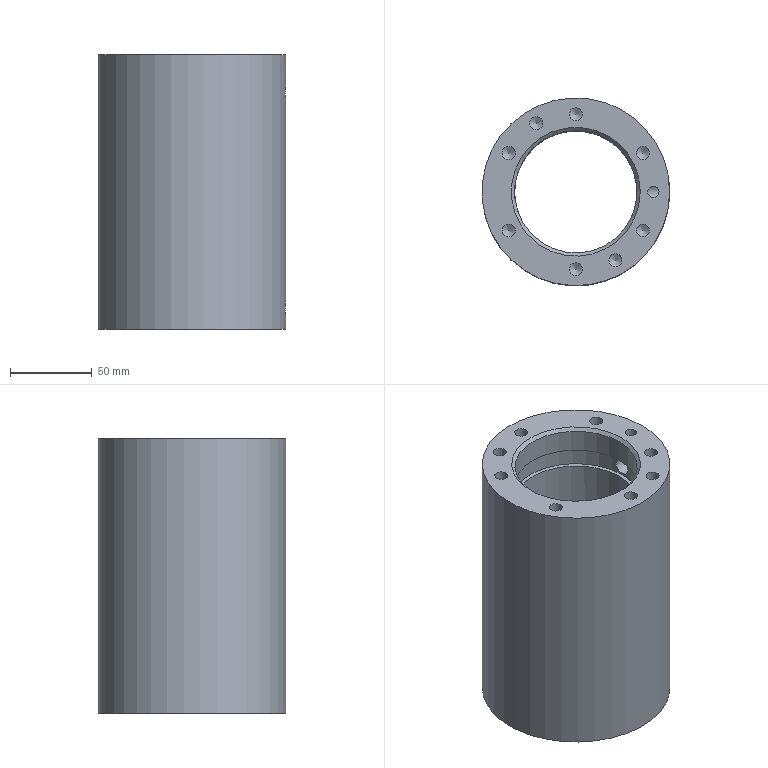Component | NX | CYLINDER_BODY | 1 solid | 52 faces | volume 967605 mm3 | cylinder 27 | cone 18 | plane 7 | commonest cylinder face diameters 8 x16 75 x3 7 x3 10 x2 80 x2 115 x1